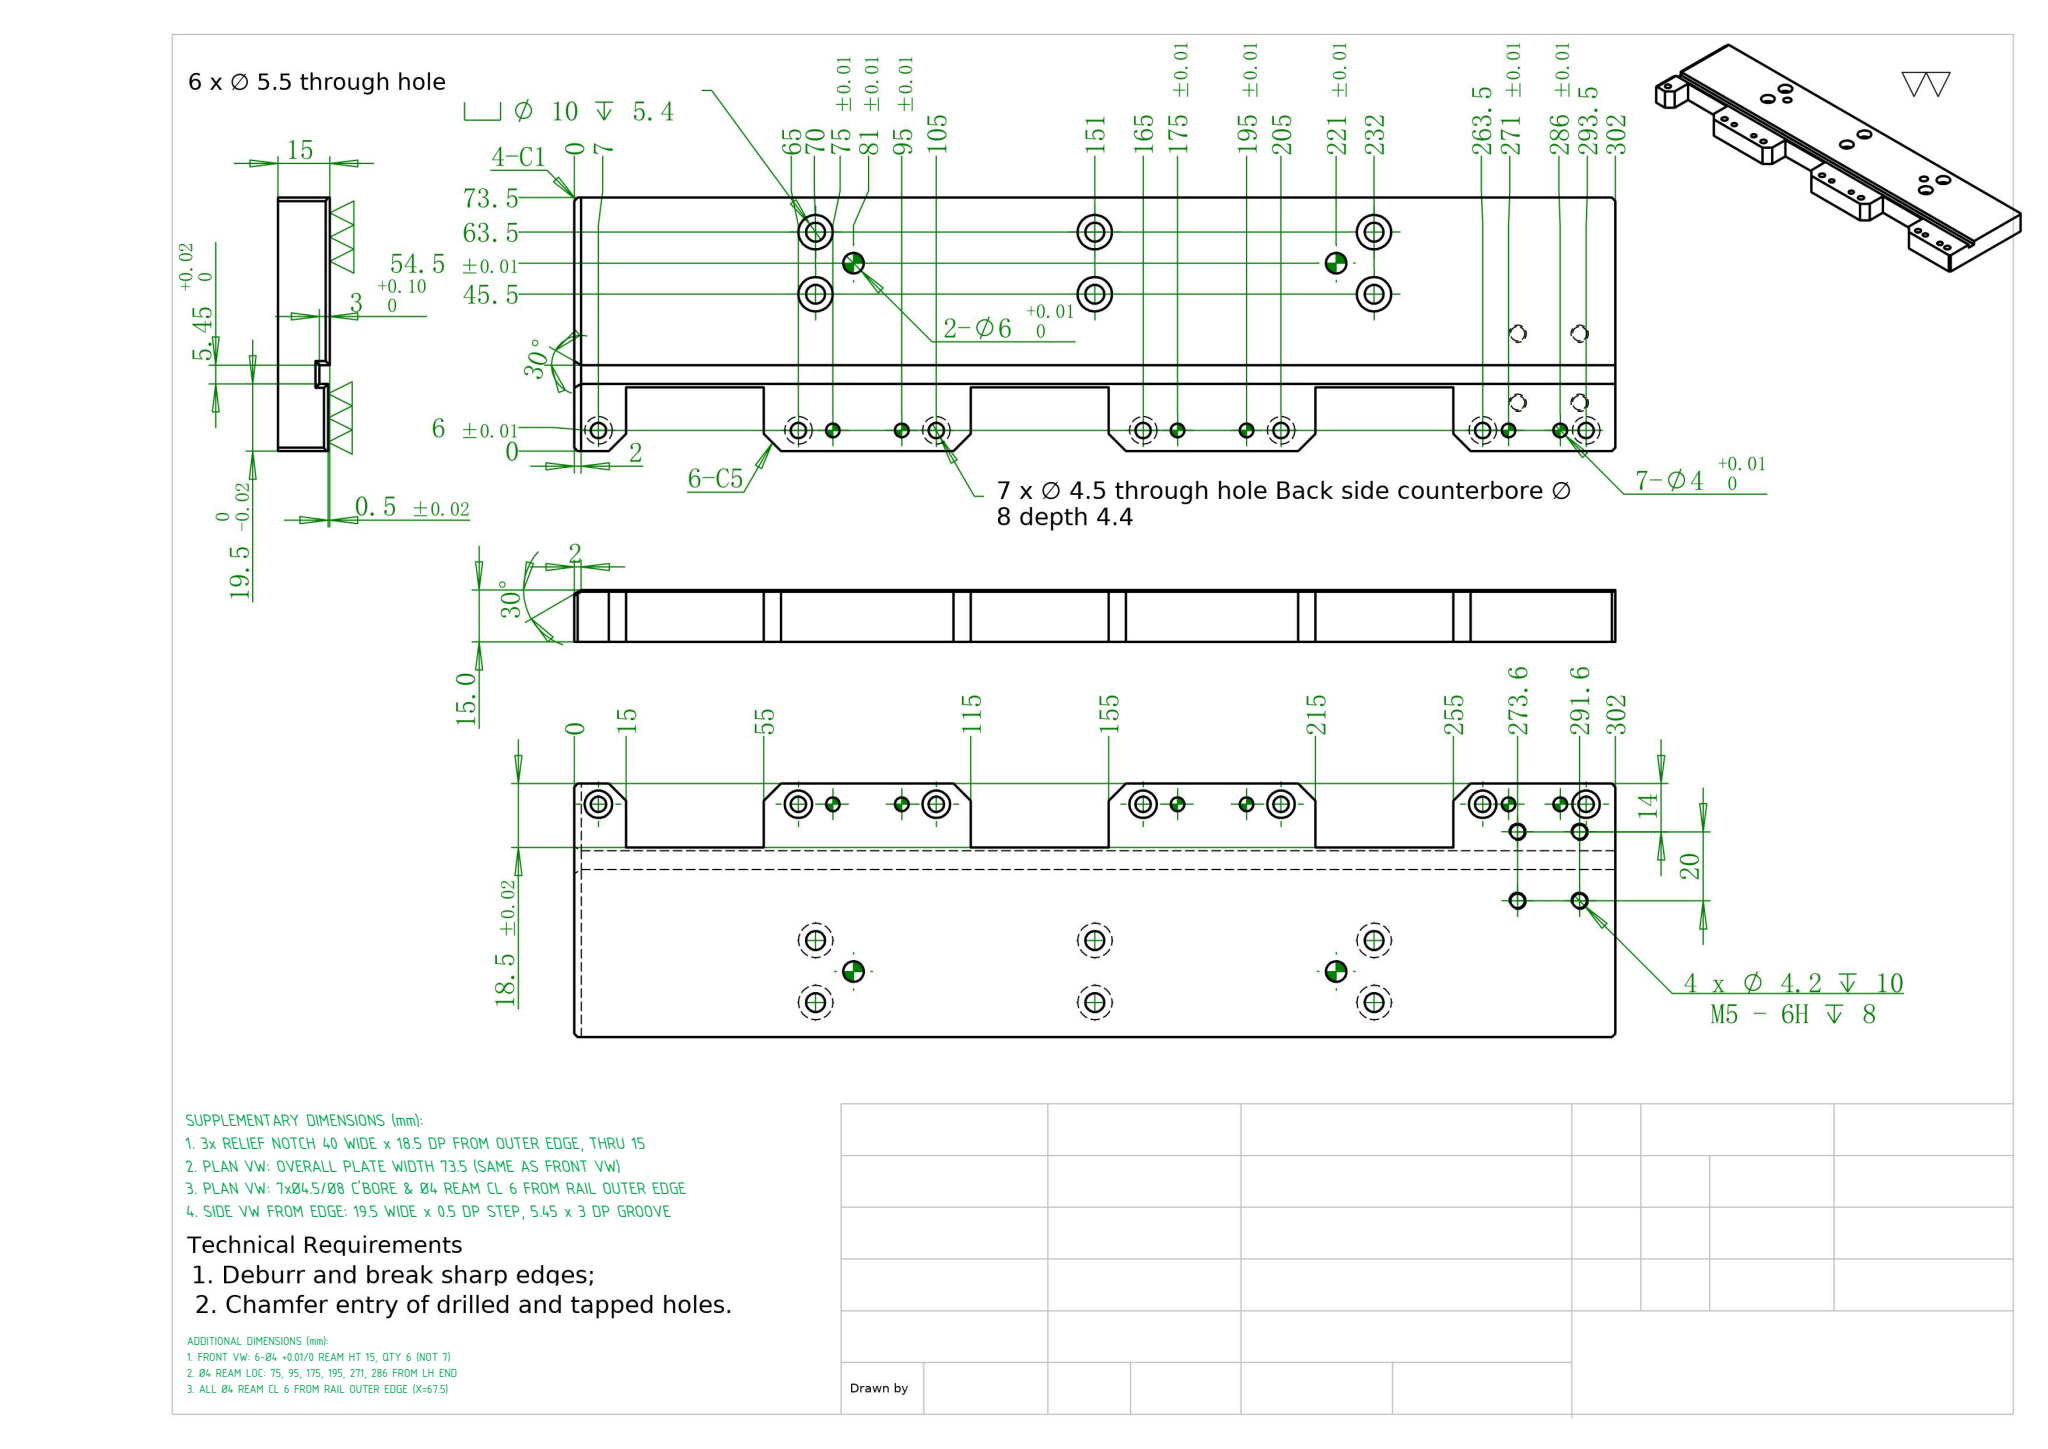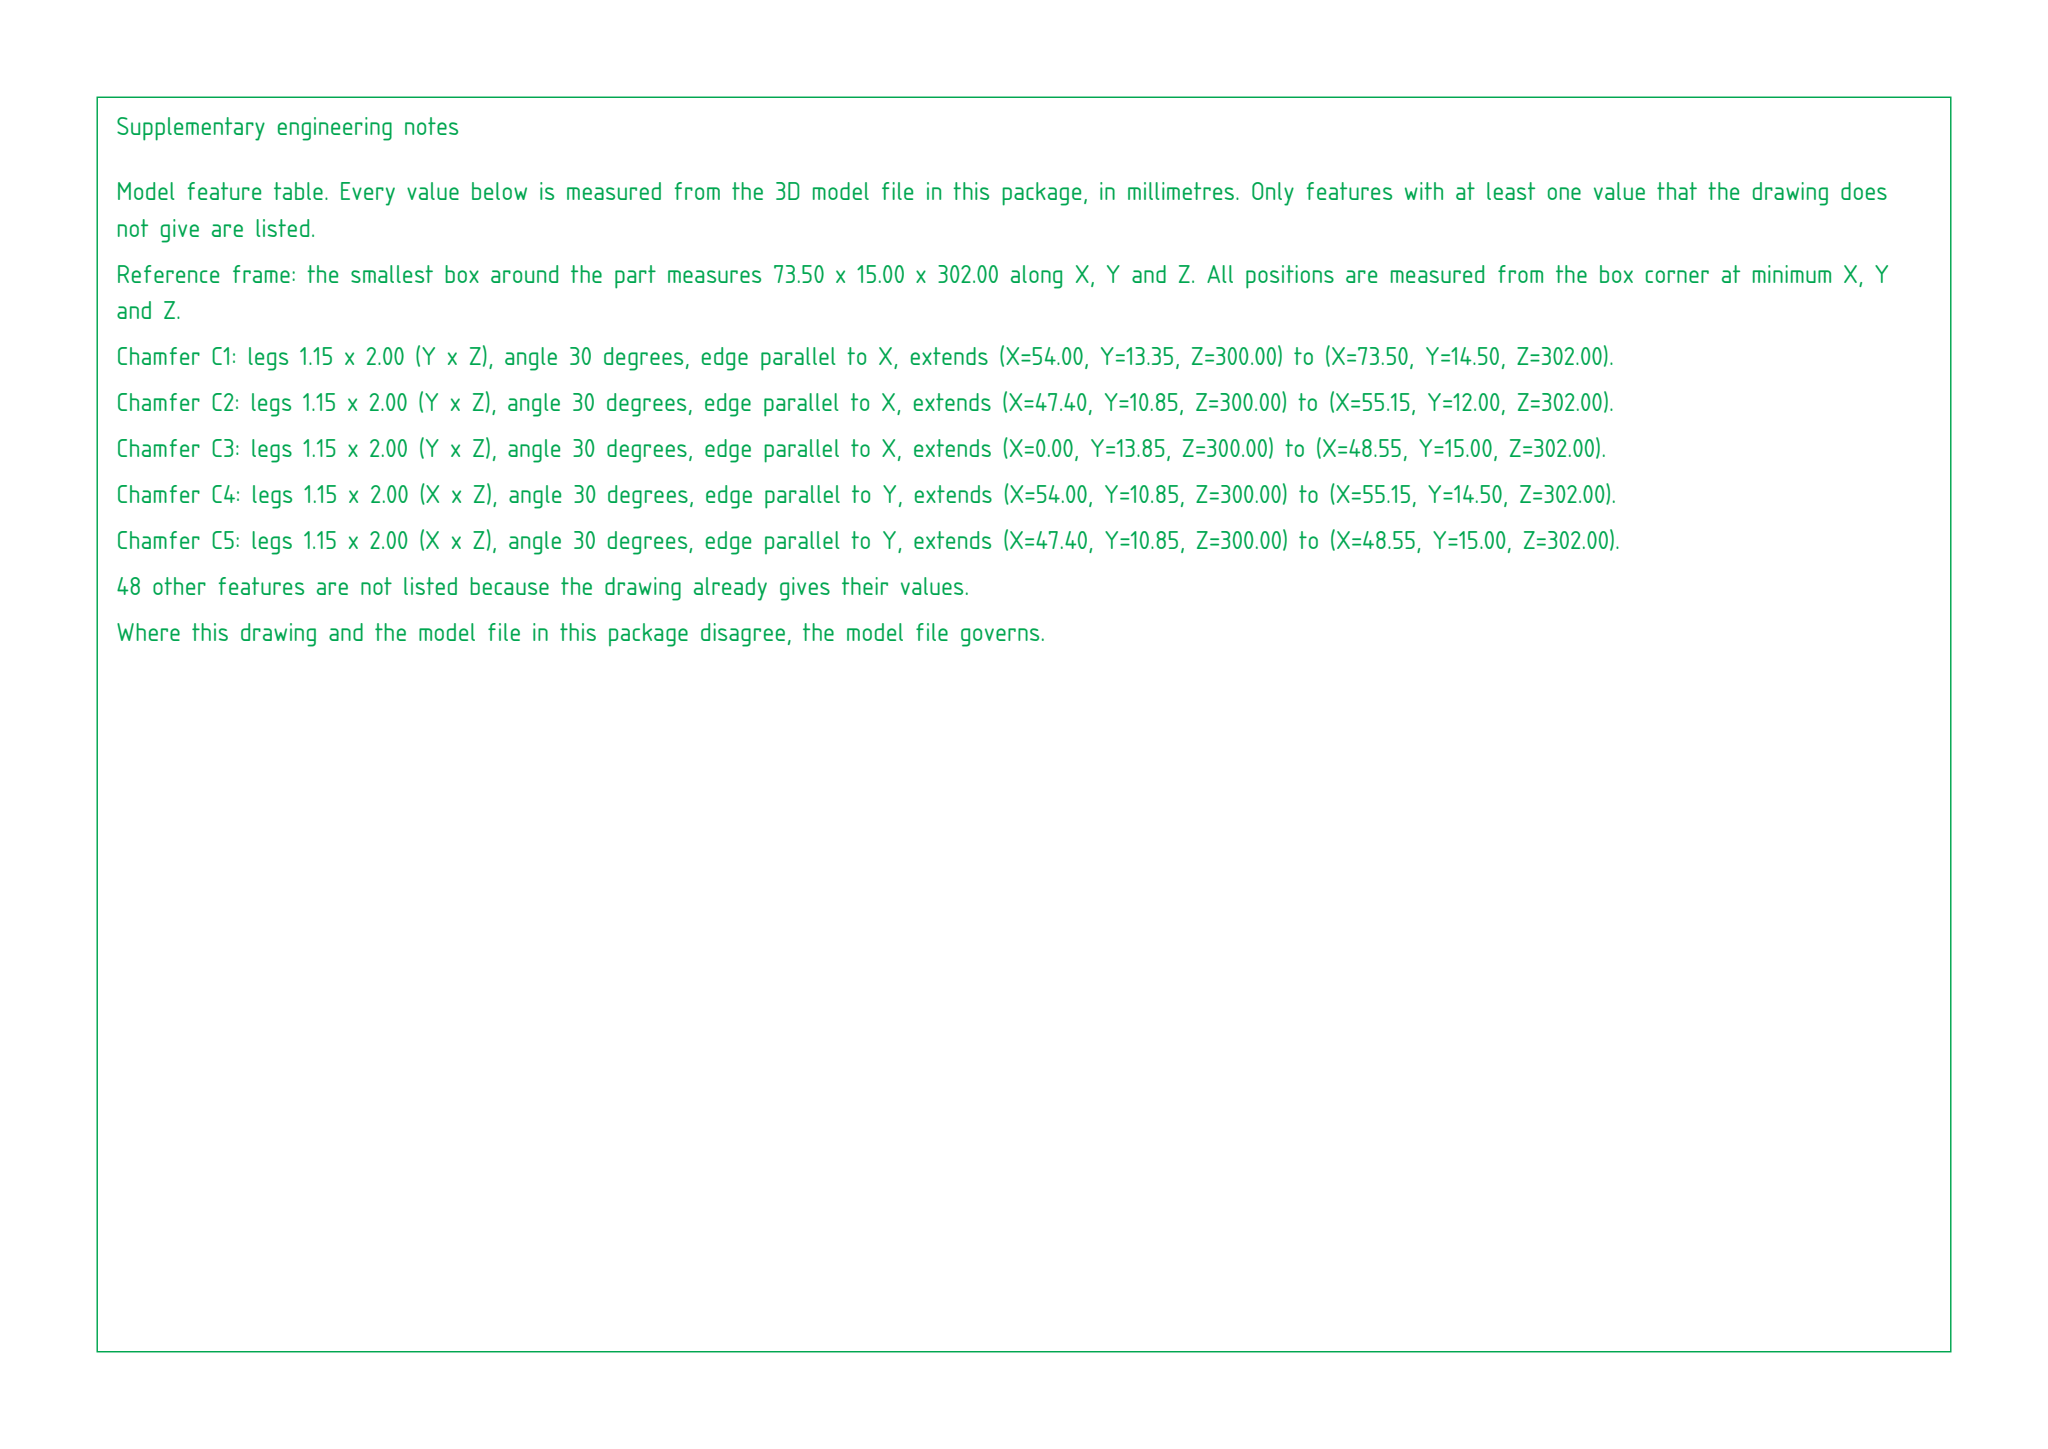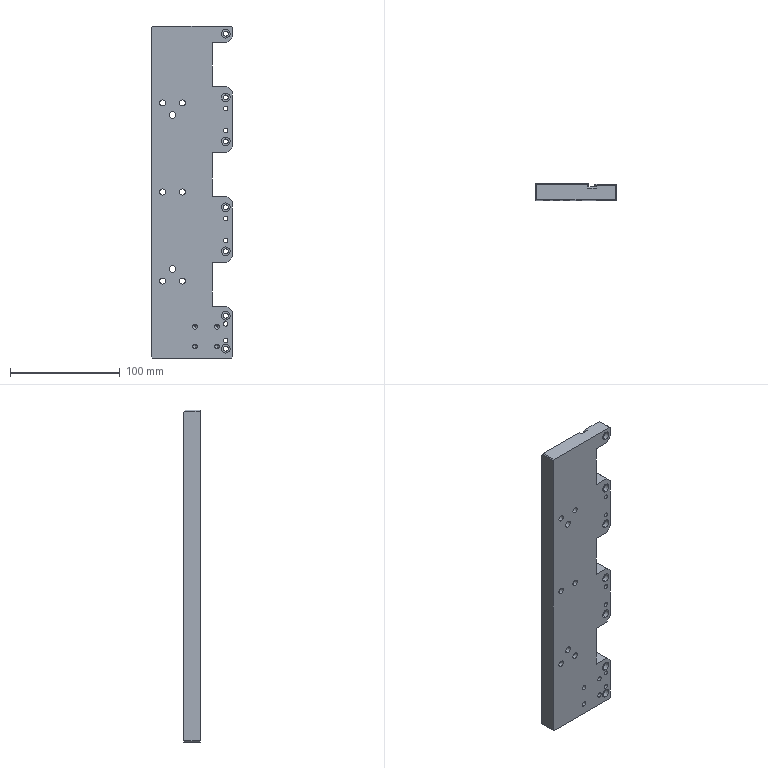Part | SolidWorks | mm | 1 solid | 134 faces | box 73.5 x 15 x 302 mm | volume 282571 mm3 | cylinder 76 | plane 50 | cone 8 | commonest cylinder face diameters 8 x14 4.5 x14 4 x12 10 x12 5.5 x12 4.2 x8 6 x4
build123d program:
from build123d import *
from OCP.BRepFilletAPI import BRepFilletAPI_MakeChamfer

# Parameters (mm, degrees)
BOSS_EXTRUDE1_DEPTH                             = 202
SKETCH2_W                                       = 19.5
SKETCH2_H                                       = 202
CUT_EXTRUDE1_DEPTH                              = 0.5
SKETCH3_W                                       = 18.5
SKETCH3_H                                       = 40
CUT_EXTRUDE2_DEPTH                              = 216.445
BOSS_EXTRUDE2_DEPTH                             = 100
LPATTERN1_COUNT                                 = 3
LPATTERN1_PITCH                                 = 100
CHAMFER1_SIZE                                   = 5
M4_HEX_SOCKET_HEAD_CAP_SCREW_CBORE1_D           = 4.5
M4_HEX_SOCKET_HEAD_CAP_SCREW_CBORE1_CBORE_D     = 8
M4_HEX_SOCKET_HEAD_CAP_SCREW_CBORE1_CBORE_DEPTH = 4.4
F_4_0_4_DIAMETER_HOLE1_D                        = 4
M5_HEX_SOCKET_HEAD_CAP_SCREW_CBORE1_D           = 5.5
M5_HEX_SOCKET_HEAD_CAP_SCREW_CBORE1_CBORE_D     = 10
M5_HEX_SOCKET_HEAD_CAP_SCREW_CBORE1_CBORE_DEPTH = 5.4
F_6_0_6_DIAMETER_HOLE1_D                        = 6
F_4_0_4_DIAMETER_HOLE2_D                        = 4
F_4_0_4_DIAMETER_HOLE2_DEPTH                    = 14.5
F_4_0_4_DIAMETER_HOLE2_TIP                      = 1.202
M5_TAPPED_HOLE1_D                               = 4.2
M5_TAPPED_HOLE1_DEPTH                           = 10
M5_TAPPED_HOLE1_TIP                             = 1.262
CHAMFER2_SIZE                                   = 2
CHAMFER2_SIZE2                                  = 1.155
CHAMFER3_SIZE                                   = 1


with BuildPart() as part:
    # Sketch1 → Boss-Extrude1 (new body)
    with BuildSketch(Plane.XY):
        Polygon((0, 0), (0, 15), (48.55, 15), (48.55, 12), (54, 12), (54, 15), (73.5, 15), (73.5, 0), align=None)
    extrude(amount=BOSS_EXTRUDE1_DEPTH)

    # Sketch2 → Cut-Extrude1 (cut)
    with BuildSketch(Plane(origin=(0, 15, 0), x_dir=(1, 0, 0), z_dir=(0, 1, 0))):
        with Locations((63.75, -101)):
            Rectangle(SKETCH2_W, SKETCH2_H)
    extrude(amount=-CUT_EXTRUDE1_DEPTH, mode=Mode.SUBTRACT)

    # Sketch3 → Cut-Extrude2 (cut, through all)
    with BuildSketch(Plane(origin=(0, 14.5, 0), x_dir=(1, 0, 0), z_dir=(0, 1, 0))):
        with Locations((64.25, -167)):
            Rectangle(SKETCH3_W, SKETCH3_H)
    cut_extrude2 = extrude(amount=-CUT_EXTRUDE2_DEPTH, mode=Mode.SUBTRACT)

    # Sketch13 → Boss-Extrude2 (add)
    with BuildSketch(Plane(origin=(0, 0, 0), x_dir=(-1, 0, 0), z_dir=(0, 0, -1))):
        Polygon((-54, 12), (-54, 14.5), (-73.5, 14.5), (-73.5, 0), (0, 0), (0, 15), (-48.55, 15), (-48.55, 12), align=None)
    extrude(amount=BOSS_EXTRUDE2_DEPTH)

    # LPattern1: Cut-Extrude2 ×3
    with Locations(*[(0, 0, -i * LPATTERN1_PITCH) for i in range(1, LPATTERN1_COUNT)]):
        add(cut_extrude2, mode=Mode.SUBTRACT)

    # Chamfer1
    chamfer1_edges = [part.edges().sort_by_distance(p)[0] for p in [
        (73.5, 7.25, 147),
        (73.5, 7.25, 187),
        (73.5, 7.25, 47),
        (73.5, 7.25, 87),
        (73.5, 7.25, -53),
        (73.5, 7.25, -13),
    ]]
    chamfer(chamfer1_edges, length=CHAMFER1_SIZE)

    # M4 Hex Socket Head Cap Screw CBORE1 (through all)
    with Locations(Plane(origin=(0, 0, 0), x_dir=(-1, 0, 0), z_dir=(0, -1, 0))):
        with Locations((-67.5, 3), (-67.5, -37), (-67.5, -97), (-67.5, -137), (-67.5, -195), (-67.5, 61.5), (-67.5, 91.5)):
            CounterBoreHole(M4_HEX_SOCKET_HEAD_CAP_SCREW_CBORE1_D / 2, M4_HEX_SOCKET_HEAD_CAP_SCREW_CBORE1_CBORE_D / 2, M4_HEX_SOCKET_HEAD_CAP_SCREW_CBORE1_CBORE_DEPTH)

    # 4.0 _4_ Diameter Hole1 (through all)
    with Locations(Plane(origin=(0, 0, 0), x_dir=(-1, 0, 0), z_dir=(0, -1, 0))):
        with Locations((-67.5, -127), (-67.5, -27), (-67.5, -7), (-67.5, -107)):
            Hole(F_4_0_4_DIAMETER_HOLE1_D / 2)

    # M5 Hex Socket Head Cap Screw CBORE1 (through all)
    with Locations(Plane(origin=(0, 15, 0), x_dir=(1, 0, 0), z_dir=(0, 1, 0))):
        with Locations((28, 30), (10, 30), (10, -132), (28, -132), (10, -51), (28, -51)):
            CounterBoreHole(M5_HEX_SOCKET_HEAD_CAP_SCREW_CBORE1_D / 2, M5_HEX_SOCKET_HEAD_CAP_SCREW_CBORE1_CBORE_D / 2, M5_HEX_SOCKET_HEAD_CAP_SCREW_CBORE1_CBORE_DEPTH)

    # 6.0 _6_ Diameter Hole1 (through all)
    with Locations(Plane(origin=(0, 15, 0), x_dir=(1, 0, 0), z_dir=(0, 1, 0))):
        with Locations((19, -121), (19, 19)):
            Hole(F_6_0_6_DIAMETER_HOLE1_D / 2)

    # 4.0 _4_ Diameter Hole2
    with Locations(Plane(origin=(0, 0, 0), x_dir=(-1, 0, 0), z_dir=(0, -1, 0))):
        with Locations((-67.5, 84), (-67.5, 69)):
            Hole(F_4_0_4_DIAMETER_HOLE2_D / 2, depth=F_4_0_4_DIAMETER_HOLE2_DEPTH)
            with Locations((0, 0, -(F_4_0_4_DIAMETER_HOLE2_DEPTH + F_4_0_4_DIAMETER_HOLE2_TIP / 2))):  # 118° drill point
                Cone(0, F_4_0_4_DIAMETER_HOLE2_D / 2, F_4_0_4_DIAMETER_HOLE2_TIP, mode=Mode.SUBTRACT)

    # M5 Tapped Hole1
    with Locations(Plane(origin=(0, 0, 0), x_dir=(-1, 0, 0), z_dir=(0, -1, 0))):
        with Locations((-39.5, 89.6), (-39.5, 71.6), (-59.5, 89.6), (-59.5, 71.6)):
            Hole(M5_TAPPED_HOLE1_D / 2, depth=M5_TAPPED_HOLE1_DEPTH)
            with Locations((0, 0, -(M5_TAPPED_HOLE1_DEPTH + M5_TAPPED_HOLE1_TIP / 2))):  # 118° drill point
                Cone(0, M5_TAPPED_HOLE1_D / 2, M5_TAPPED_HOLE1_TIP, mode=Mode.SUBTRACT)

    # Chamfer2: one chamfer whose edges measure the first distance from different faces: ONE call of the kernel's chamfer builder (chamfer() names one face for all edges)
    chamfer2_edges_1 = [part.edges().sort_by_distance(p)[0] for p in [
        (51.275, 12, 202),
    ]]
    chamfer2_side_1 = [part.faces().sort_by_distance(p)[0] for p in [
        (51.275, 12, 51),
    ]]
    chamfer2_edges_2 = [part.edges().sort_by_distance(p)[0] for p in [
        (48.55, 13.5, 202),
    ]]
    chamfer2_side_2 = [part.faces().sort_by_distance(p)[0] for p in [
        (48.55, 13.5, 51),
    ]]
    chamfer2_edges_3 = [part.edges().sort_by_distance(p)[0] for p in [
        (24.275, 15, 202),
    ]]
    chamfer2_side_3 = [part.faces().sort_by_distance(p)[0] for p in [
        (3.059, 15, 51),
    ]]
    chamfer2_edges_4 = [part.edges().sort_by_distance(p)[0] for p in [
        (54, 13.25, 202),
    ]]
    chamfer2_side_4 = [part.faces().sort_by_distance(p)[0] for p in [
        (54, 13.25, 51),
    ]]
    chamfer2_edges_5 = [part.edges().sort_by_distance(p)[0] for p in [
        (63.75, 14.5, 202),
    ]]
    chamfer2_side_5 = [part.faces().sort_by_distance(p)[0] for p in [
        (63.041, 14.5, 41.147),
    ]]
    chamfer2 = BRepFilletAPI_MakeChamfer(part.part.solid().wrapped)
    for e in chamfer2_edges_1:
        chamfer2.Add(CHAMFER2_SIZE, CHAMFER2_SIZE2, e.wrapped, chamfer2_side_1[0].wrapped)  # the first distance lies on this face
    for e in chamfer2_edges_2:
        chamfer2.Add(CHAMFER2_SIZE, CHAMFER2_SIZE2, e.wrapped, chamfer2_side_2[0].wrapped)  # the first distance lies on this face
    for e in chamfer2_edges_3:
        chamfer2.Add(CHAMFER2_SIZE, CHAMFER2_SIZE2, e.wrapped, chamfer2_side_3[0].wrapped)  # the first distance lies on this face
    for e in chamfer2_edges_4:
        chamfer2.Add(CHAMFER2_SIZE, CHAMFER2_SIZE2, e.wrapped, chamfer2_side_4[0].wrapped)  # the first distance lies on this face
    for e in chamfer2_edges_5:
        chamfer2.Add(CHAMFER2_SIZE, CHAMFER2_SIZE2, e.wrapped, chamfer2_side_5[0].wrapped)  # the first distance lies on this face
    add(Compound.cast(chamfer2.Shape()), mode=Mode.REPLACE)

    # Chamfer3
    chamfer3_edges = [part.edges().sort_by_distance(p)[0] for p in [
        (0, 6.923, 202),
        (73.5, 7.25, -100),
        (0, 7.5, -100),
        (73.5, 6.673, 202),
    ]]
    chamfer(chamfer3_edges, length=CHAMFER3_SIZE)


solid = part.part